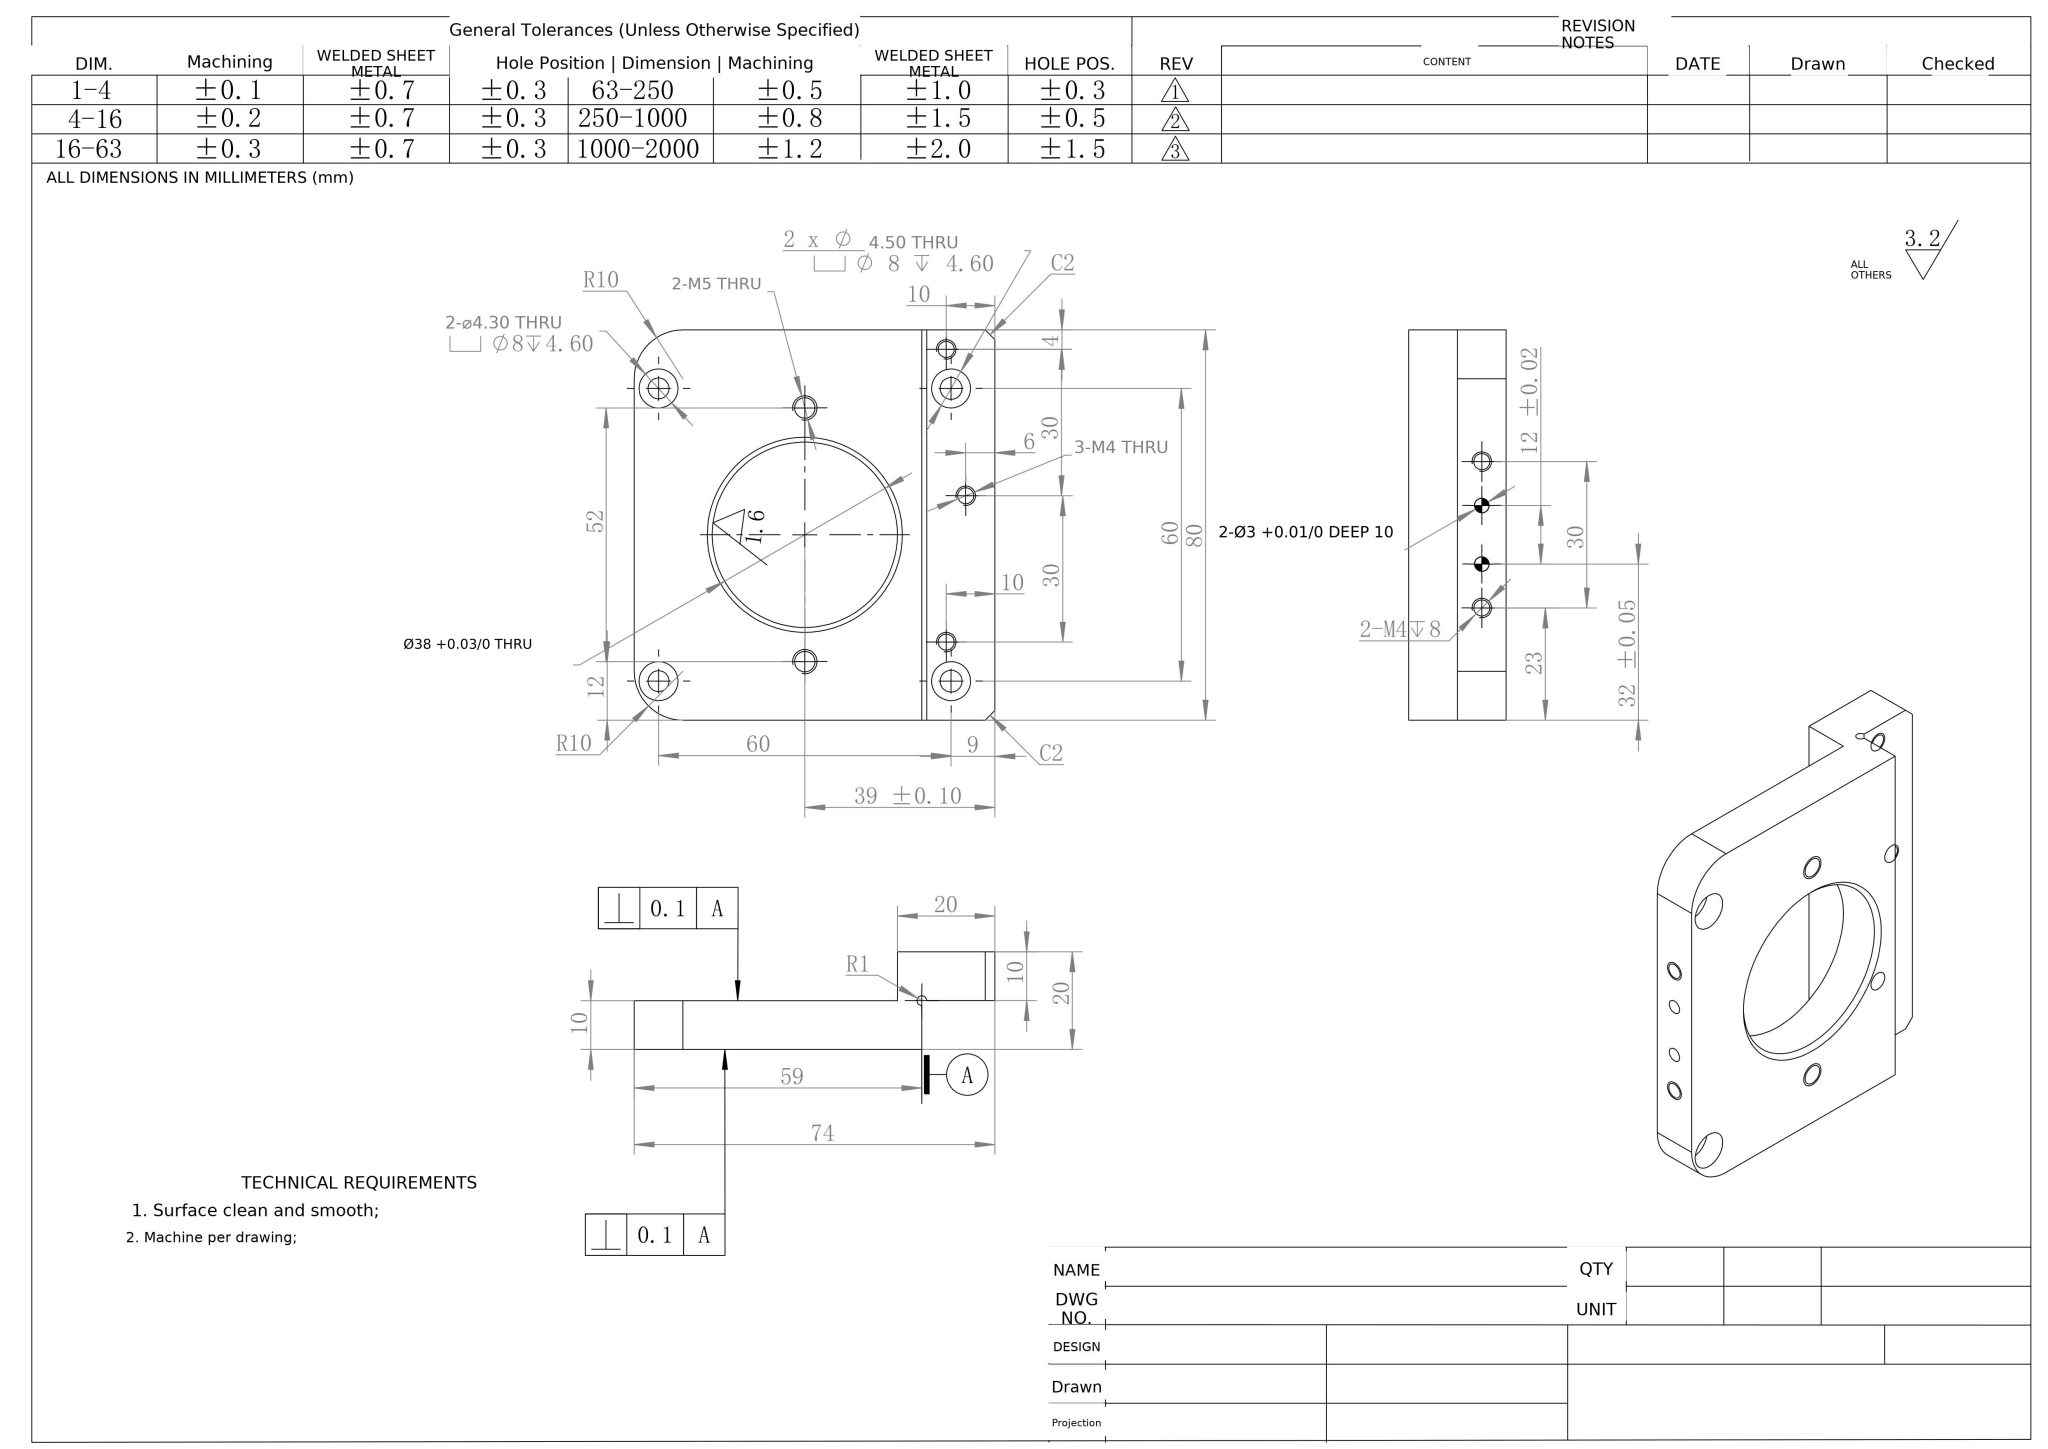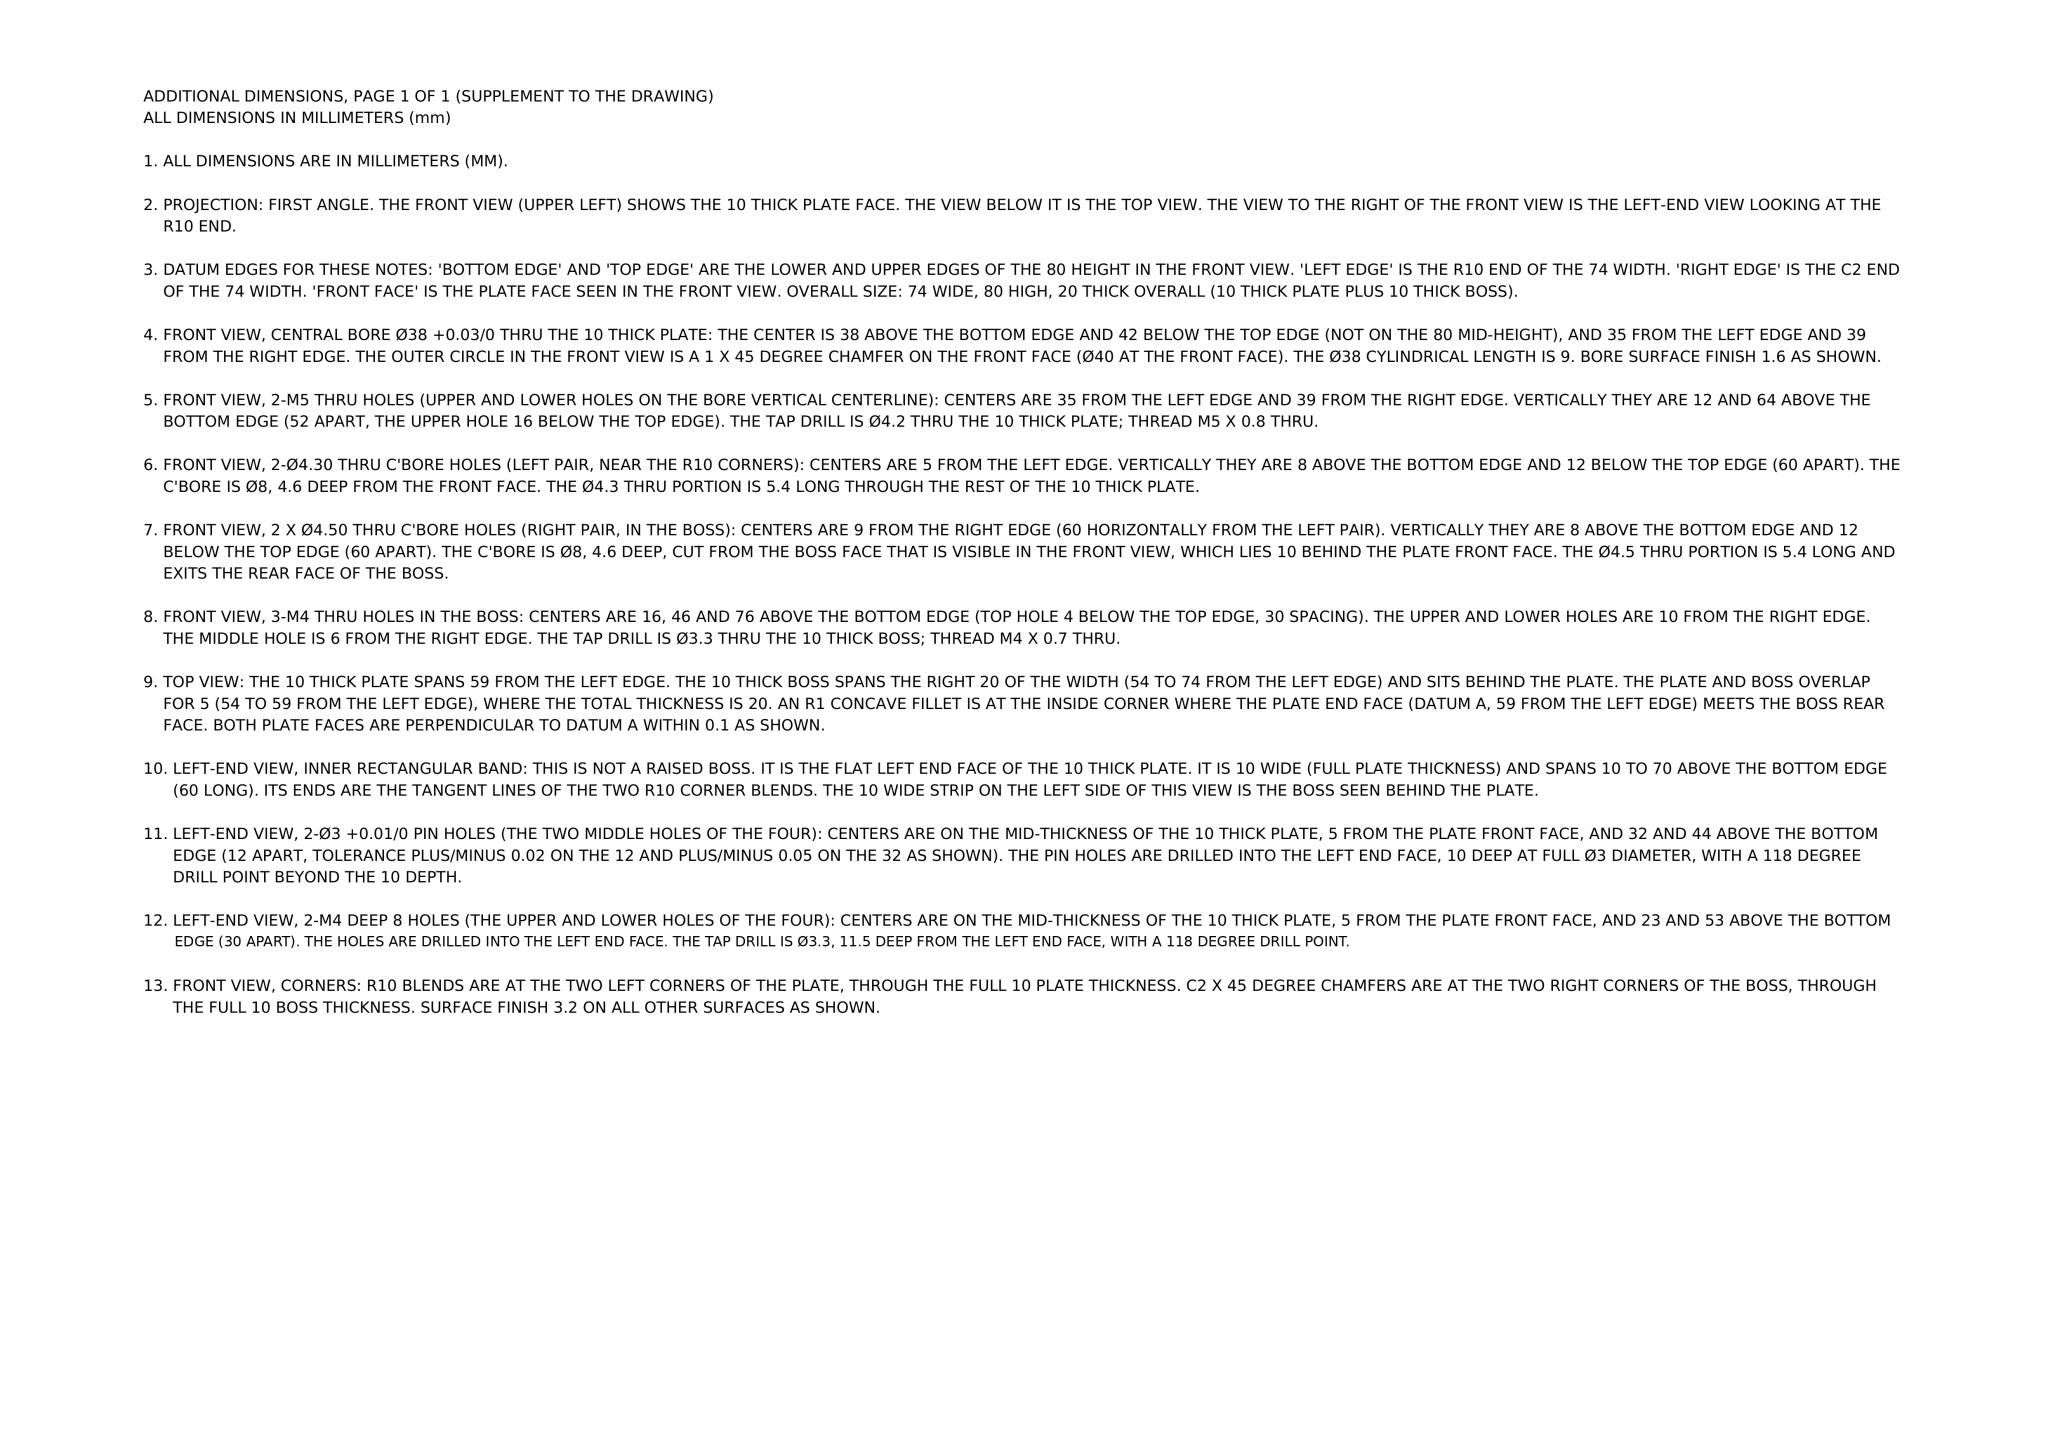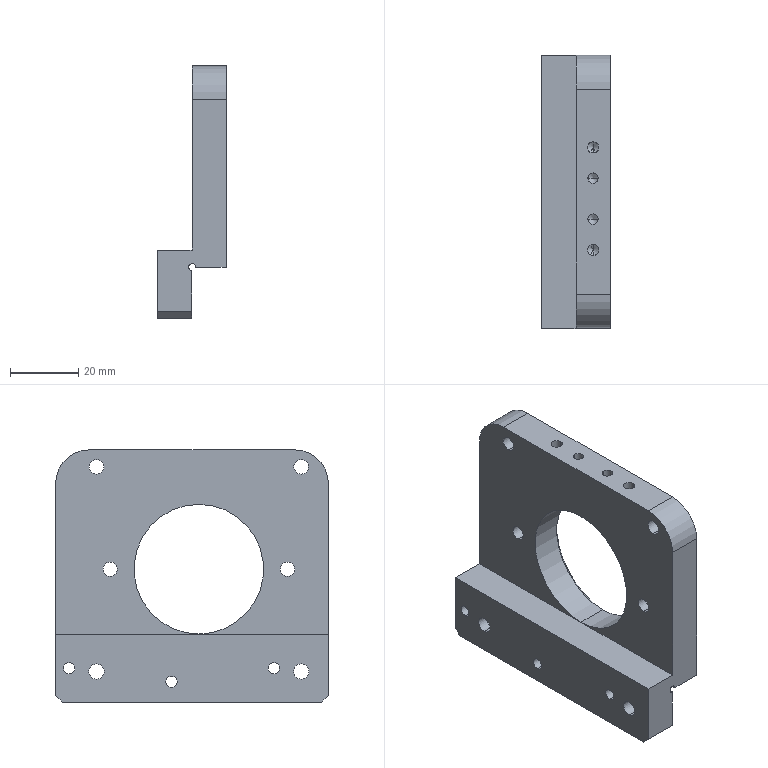Part | NX | mm | 1 solid | 66 faces | box 20 x 80 x 74 mm | volume 48987 mm3 | cylinder 40 | plane 16 | cone 10 | commonest cylinder face diameters 3.3 x10 8 x8 4.5 x4 4.2 x4 4.3 x4 3 x4 2 x2 38 x2